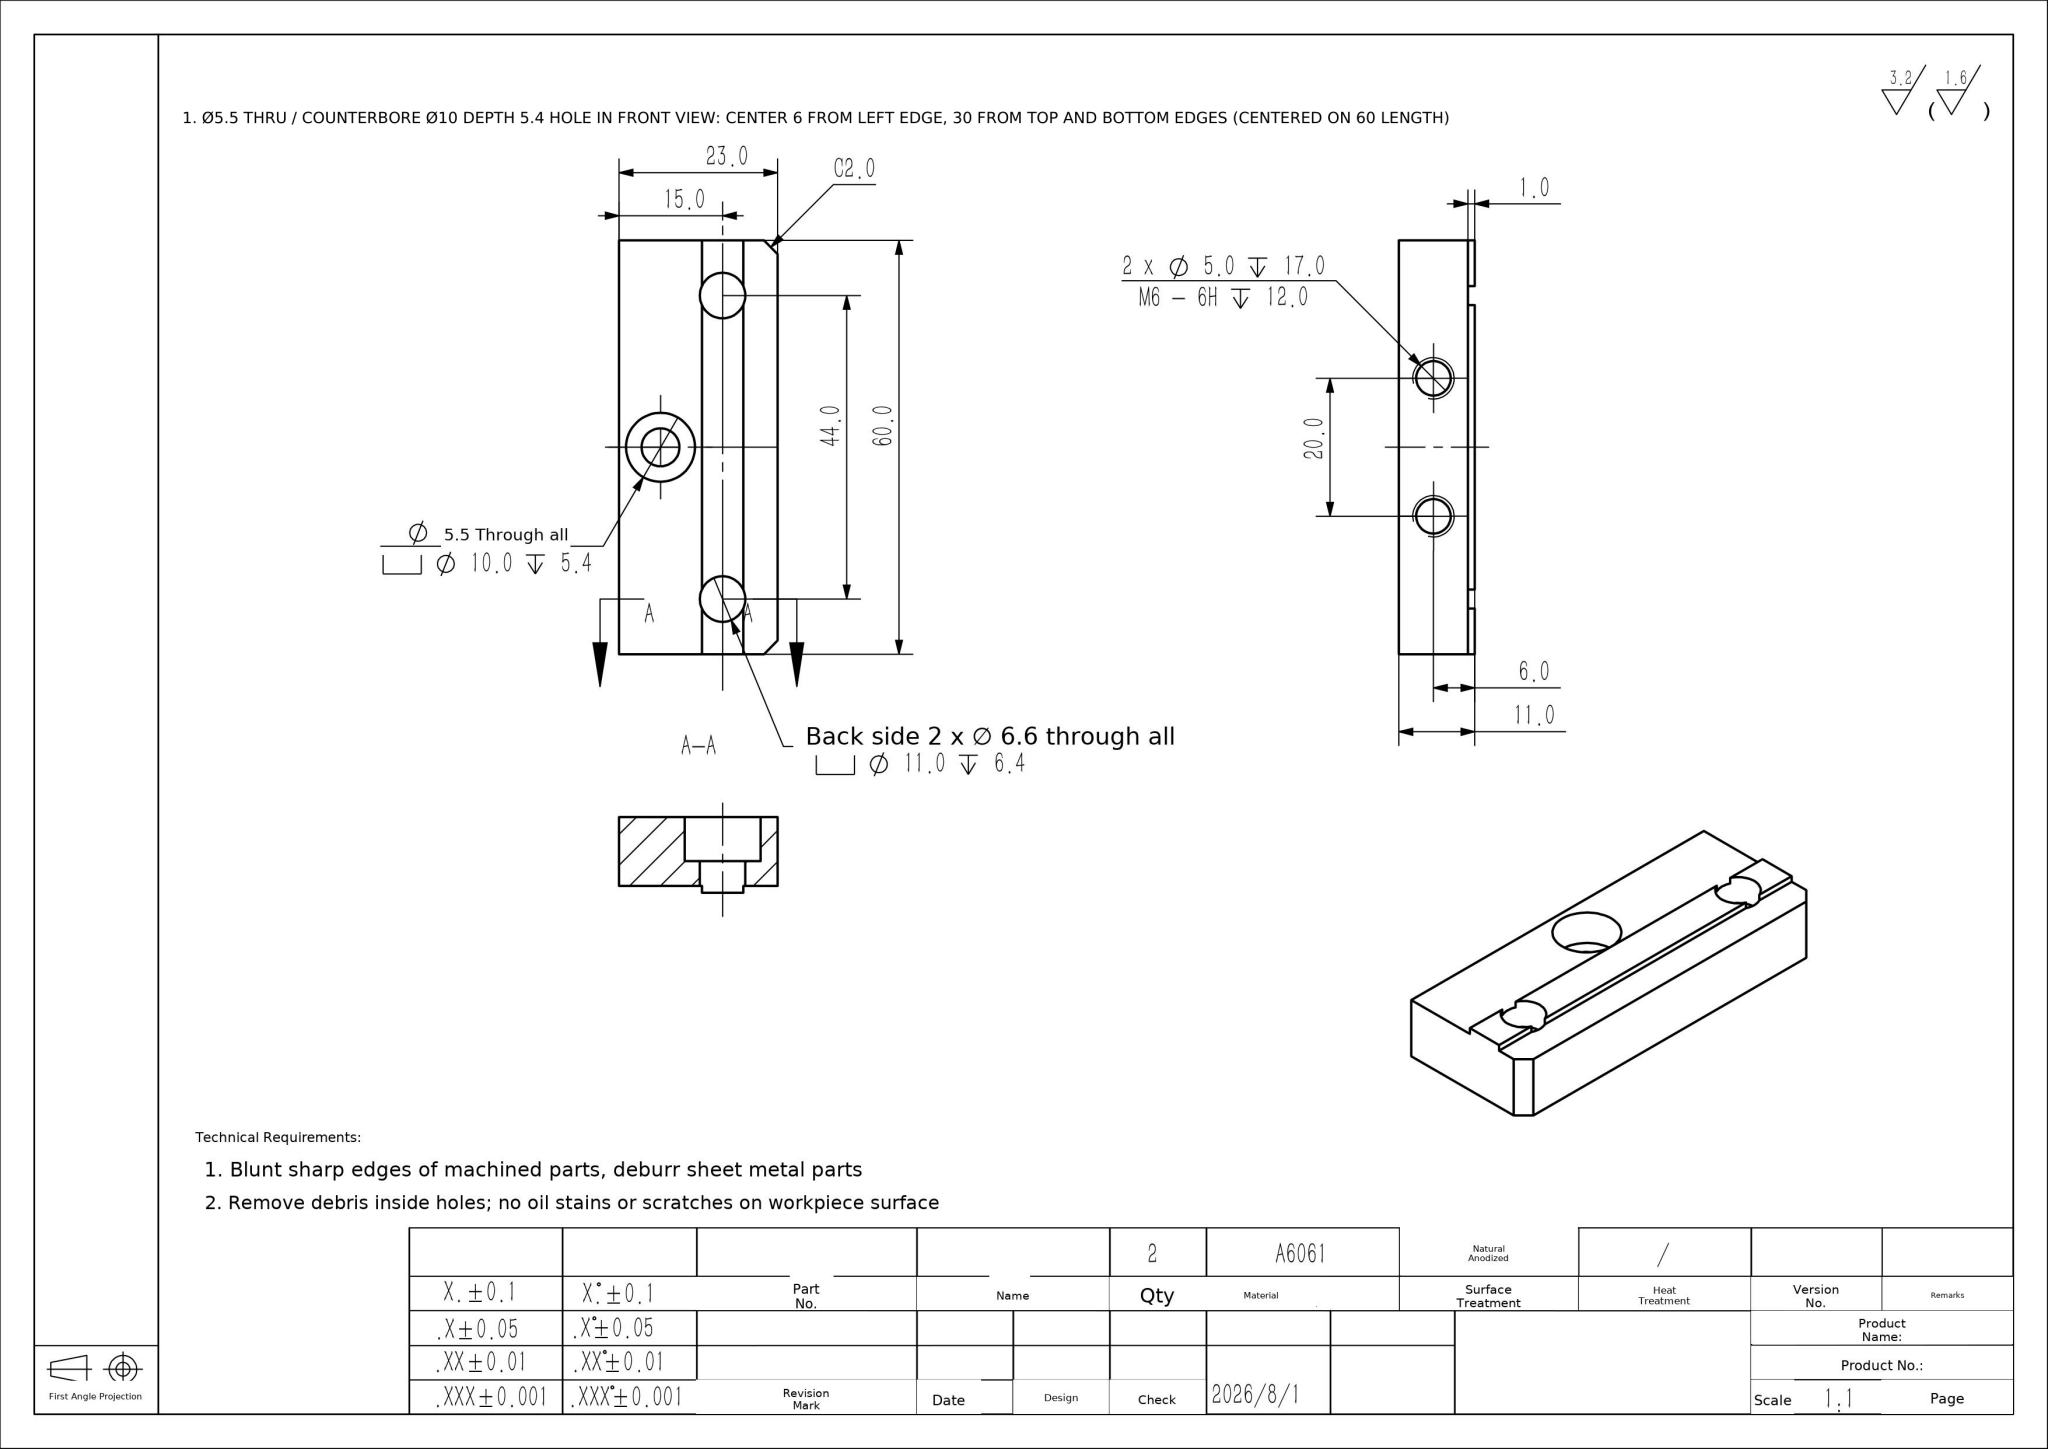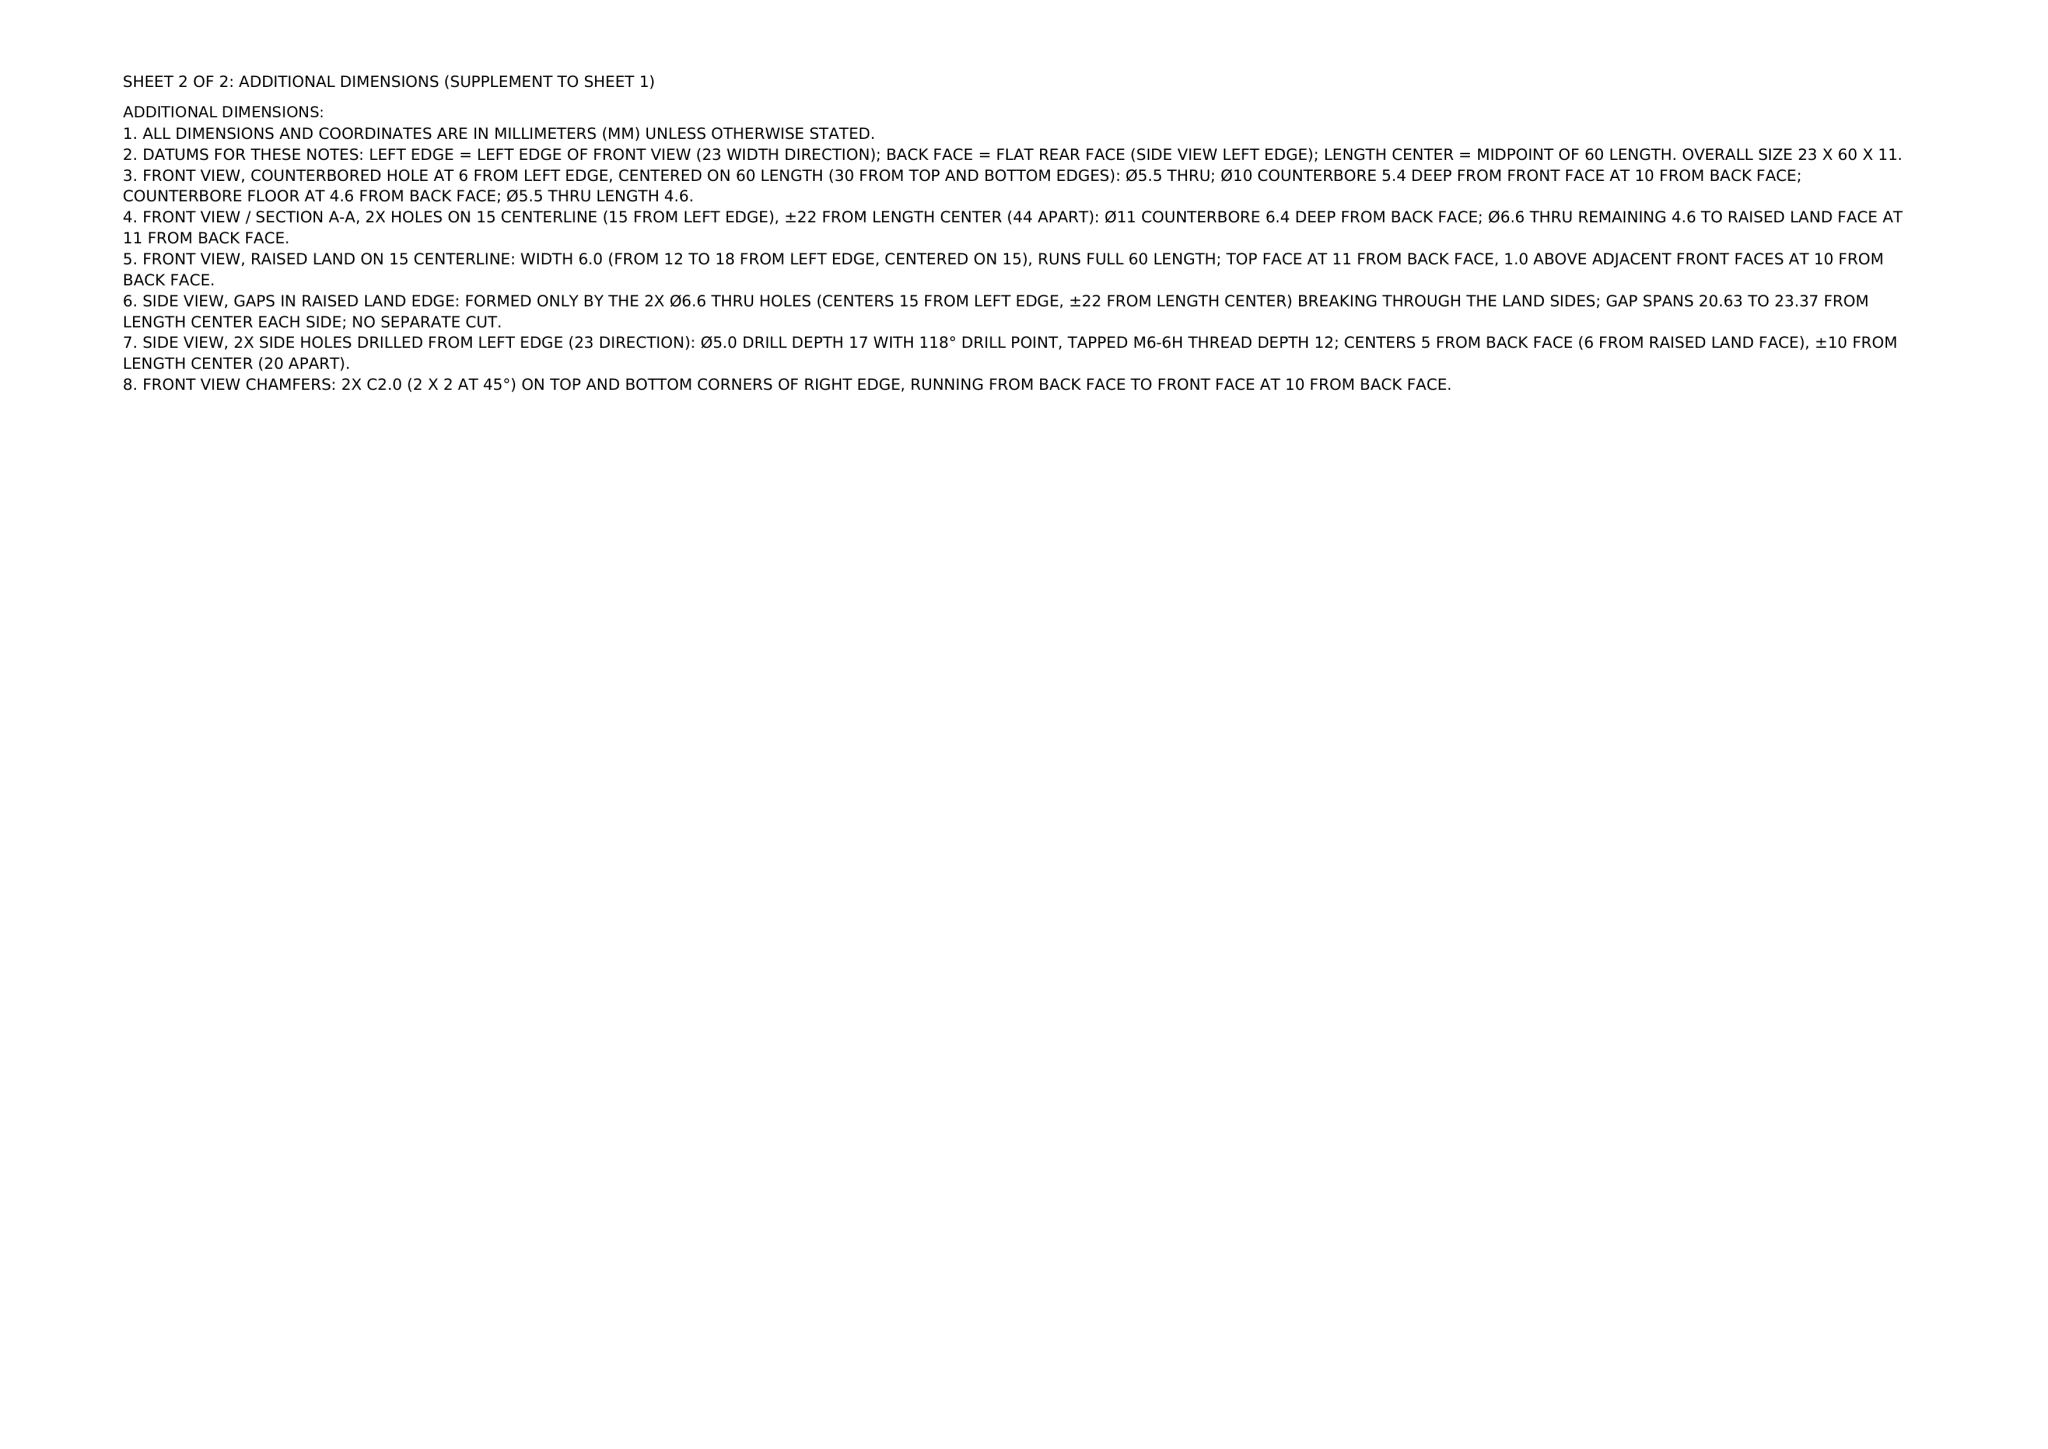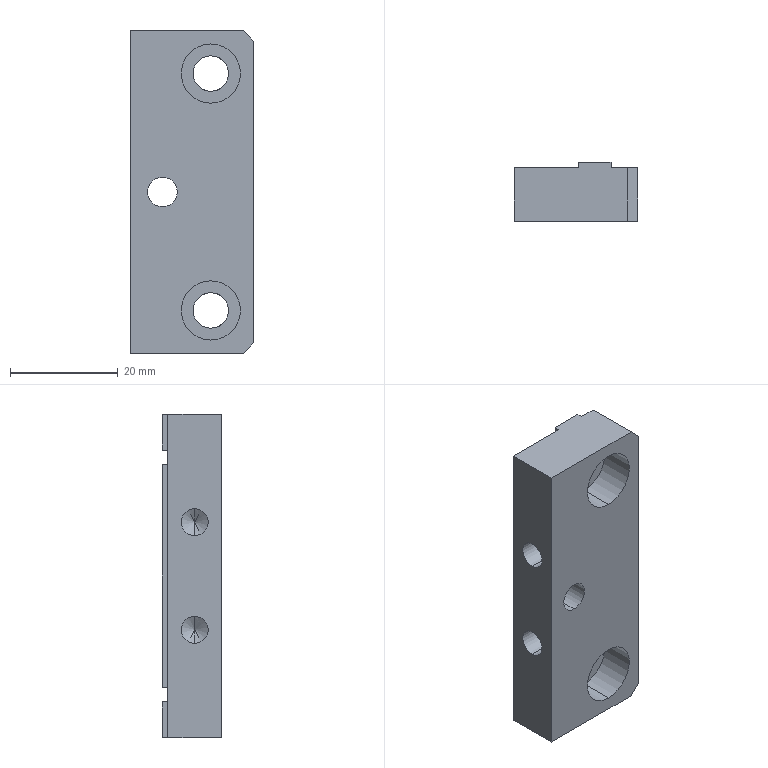Part | NX | mm | 1 solid | 41 faces | box 23 x 11 x 60 mm | volume 11370 mm3 | plane 21 | cylinder 16 | cone 4 | commonest cylinder face diameters 5 x4 11 x4 6.6 x4 10 x2 5.5 x2